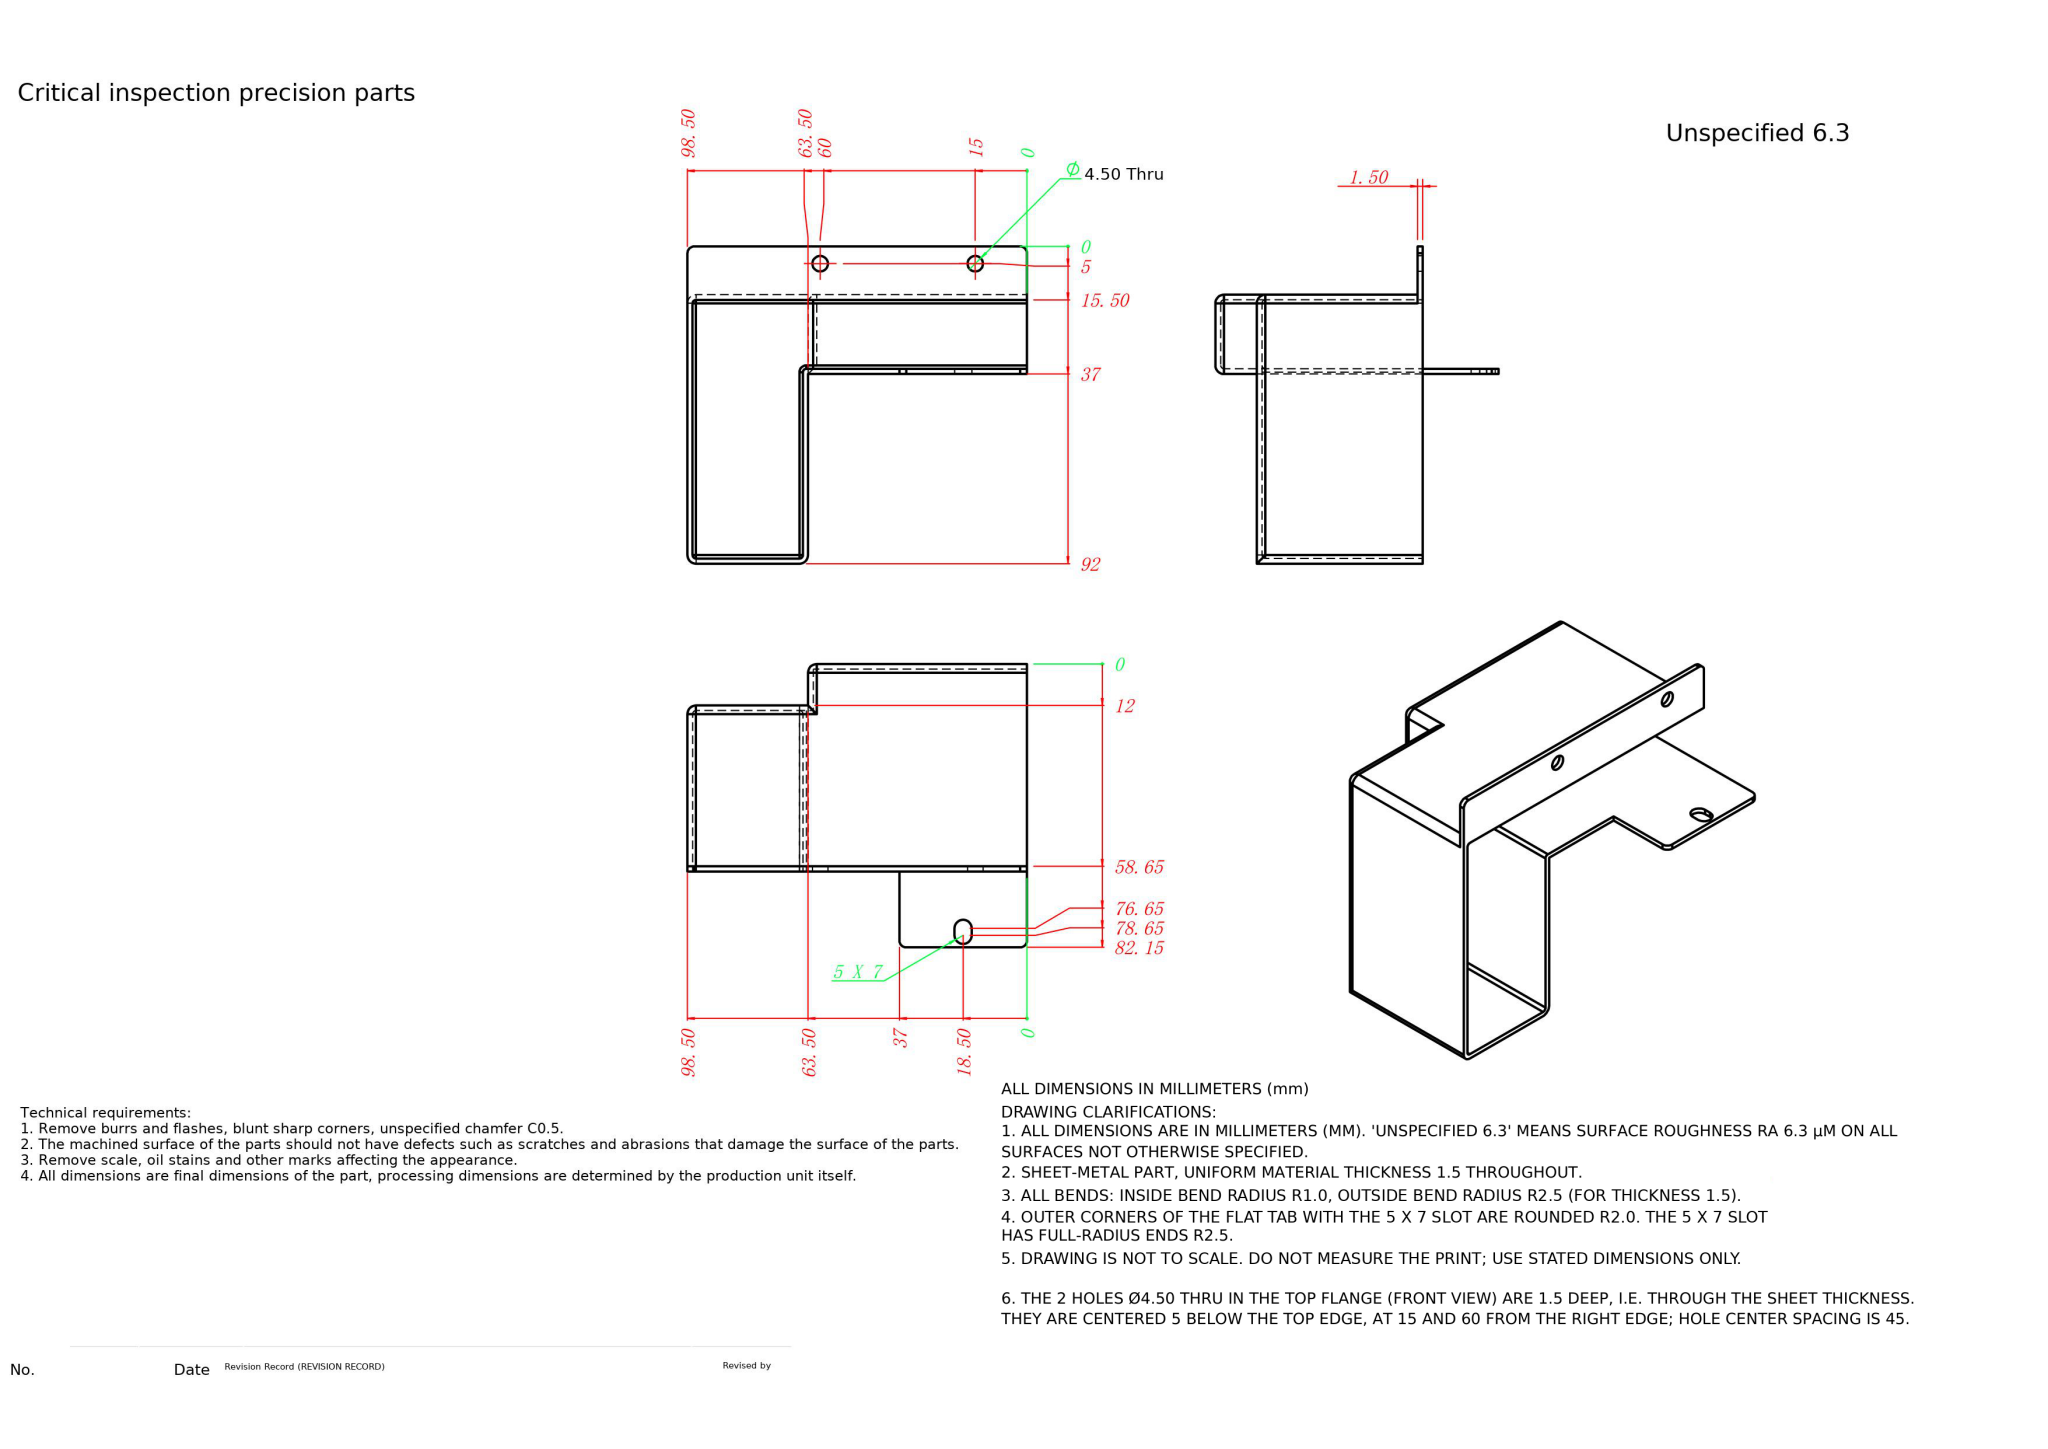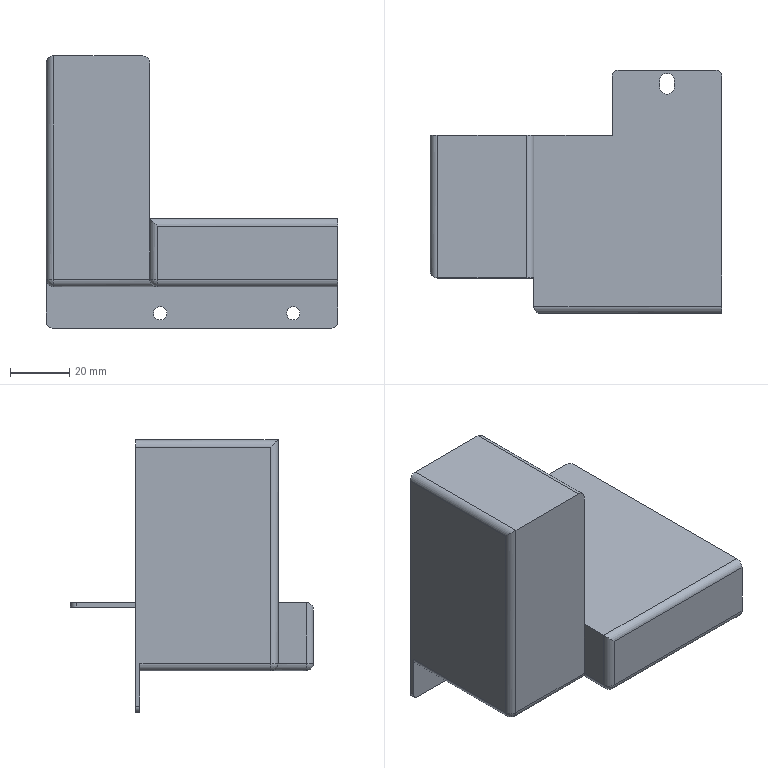Part | NX | mm | L-Shaped Tubular Mounting Bracket With Tab | 1 solid | 60 faces | box 98.5 x 82.15 x 92 mm | volume 34541 mm3 | cylinder 30 | plane 24 | sphere 5 | torus 1 | commonest cylinder face diameters 2 x11 5 x11 4.5 x4 4 x4